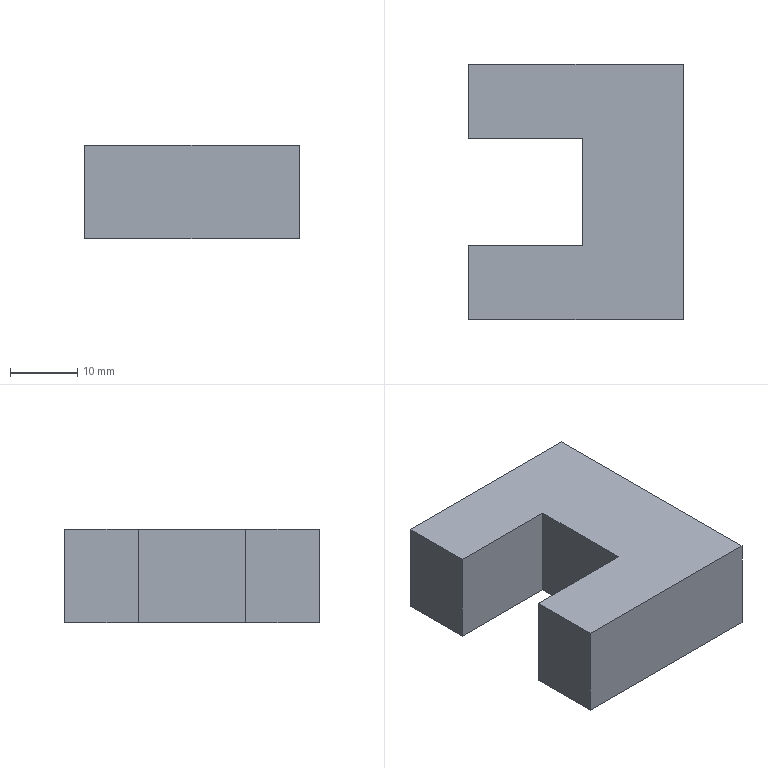Component | SolidWorks | PointedHeadDispensingStopPoint-1 | 1 solid | 18 faces | box 32 x 38 x 14 mm | volume 12816 mm3 | plane 10 | cone 4 | cylinder 4 | commonest cylinder face diameters 4.2 x4
build123d program:
from build123d import *

# Parameters (mm, degrees)
SKETCH1_W             = 32
SKETCH1_H             = 14
EXTRUDE1_DEPTH        = 38
SKETCH3_W             = 17
SKETCH3_H             = 16
CUT_EXTRUDE1_DEPTH    = 52.614
M5_TAPPED_HOLE1_D     = 4.2
M5_TAPPED_HOLE1_DEPTH = 14
M5_TAPPED_HOLE1_TIP   = 1.262


with BuildPart() as part:
    # Sketch1 → Extrude1 (new body)
    with BuildSketch(Plane(origin=(0, 0, 0), x_dir=(1, 0, 0), z_dir=(0, 1, 0))):
        with Locations((16, -7)):
            Rectangle(SKETCH1_W, SKETCH1_H)
    extrude(amount=EXTRUDE1_DEPTH)

    # Sketch3 → Cut-Extrude1 (cut, through all)
    with BuildSketch(Plane.XY.offset(14)):
        with Locations((8.5, 19)):
            Rectangle(SKETCH3_W, SKETCH3_H)
    extrude(amount=-CUT_EXTRUDE1_DEPTH, mode=Mode.SUBTRACT)

    # M5 Tapped Hole1
    with Locations(Plane(origin=(32, 0, 0), x_dir=(0, 0, -1), z_dir=(1, 0, 0))):
        with Locations((-7, 5), (-7, 33)):
            Hole(M5_TAPPED_HOLE1_D / 2, depth=M5_TAPPED_HOLE1_DEPTH)
            with Locations((0, 0, -(M5_TAPPED_HOLE1_DEPTH + M5_TAPPED_HOLE1_TIP / 2))):  # 118° drill point
                Cone(0, M5_TAPPED_HOLE1_D / 2, M5_TAPPED_HOLE1_TIP, mode=Mode.SUBTRACT)


solid = part.part

# Placed as in the assembly
solid = solid.moved(Location((-19.083, 26.872, -124.387), (0, 0, 0)))
STEP:
#1=COLOUR_RGB('',0.7922,0.8196,0.9333);
#2=FILL_AREA_STYLE_COLOUR('',#1);
#3=FILL_AREA_STYLE('',(#2));
#4=SURFACE_STYLE_FILL_AREA(#3);
#5=SURFACE_SIDE_STYLE('',(#4));
#6=SURFACE_STYLE_USAGE(.BOTH.,#5);
#7=PRESENTATION_STYLE_ASSIGNMENT((#6));
#8=CARTESIAN_POINT('',(-0.09232,1.255,-4.622));
#9=VERTEX_POINT('',#8);
#10=CARTESIAN_POINT('',(-0.04264,1.255,-4.704));
#11=VERTEX_POINT('',#10);
#12=CARTESIAN_POINT('',(-0.04264,1.255,-4.704));
#13=DIRECTION('',(0.515,0.,-0.8572));
#14=VECTOR('',#13,39.37);
#15=LINE('',#12,#14);
#16=EDGE_CURVE('',#9,#11,#15,.T.);
#17=ORIENTED_EDGE('',*,*,#16,.F.);
#18=CARTESIAN_POINT('',(-0.04264,1.255,-4.539));
#19=VERTEX_POINT('',#18);
#20=CARTESIAN_POINT('',(-0.04264,1.255,-4.539));
#21=DIRECTION('',(0.515,0.,0.8572));
#22=VECTOR('',#21,39.37);
#23=LINE('',#20,#22);
#24=EDGE_CURVE('',#9,#19,#23,.T.);
#25=ORIENTED_EDGE('',*,*,#24,.T.);
#26=CARTESIAN_POINT('',(-0.04264,1.255,-4.622));
#27=DIRECTION('',(1.,0.,0.));
#28=DIRECTION('',(0.,0.,-1.));
#29=AXIS2_PLACEMENT_3D('',#26,#27,#28);
#30=CIRCLE('',#29,0.08268);
#31=EDGE_CURVE('',#19,#11,#30,.T.);
#32=ORIENTED_EDGE('',*,*,#31,.T.);
#33=EDGE_LOOP('',(#17,#25,#32));
#34=FACE_OUTER_BOUND('',#33,.T.);
#35=CARTESIAN_POINT('',(-0.04264,1.255,-4.622));
#36=DIRECTION('',(1.,0.,0.));
#37=DIRECTION('',(0.,0.,-1.));
#38=AXIS2_PLACEMENT_3D('',#35,#36,#37);
#39=CONICAL_SURFACE('',#38,0.08268,1.03);
#40=ADVANCED_FACE('',(#34),#39,.F.);
#41=ORIENTED_EDGE('',*,*,#31,.F.);
#42=CARTESIAN_POINT('',(0.5085,1.255,-4.539));
#43=VERTEX_POINT('',#42);
#44=CARTESIAN_POINT('',(0.5085,1.255,-4.539));
#45=DIRECTION('',(1.,0.,0.));
#46=VECTOR('',#45,39.37);
#47=LINE('',#44,#46);
#48=EDGE_CURVE('',#19,#43,#47,.T.);
#49=ORIENTED_EDGE('',*,*,#48,.T.);
#50=CARTESIAN_POINT('',(0.5085,1.255,-4.704));
#51=VERTEX_POINT('',#50);
#52=CARTESIAN_POINT('',(0.5085,1.255,-4.622));
#53=DIRECTION('',(1.,0.,0.));
#54=DIRECTION('',(0.,0.,-1.));
#55=AXIS2_PLACEMENT_3D('',#52,#53,#54);
#56=CIRCLE('',#55,0.08268);
#57=EDGE_CURVE('',#43,#51,#56,.T.);
#58=ORIENTED_EDGE('',*,*,#57,.T.);
#59=CARTESIAN_POINT('',(0.5085,1.255,-4.704));
#60=DIRECTION('',(1.,0.,0.));
#61=VECTOR('',#60,39.37);
#62=LINE('',#59,#61);
#63=EDGE_CURVE('',#11,#51,#62,.T.);
#64=ORIENTED_EDGE('',*,*,#63,.F.);
#65=EDGE_LOOP('',(#41,#49,#58,#64));
#66=FACE_OUTER_BOUND('',#65,.T.);
#67=CARTESIAN_POINT('',(0.5085,1.255,-4.622));
#68=DIRECTION('',(1.,0.,0.));
#69=DIRECTION('',(0.,0.,-1.));
#70=AXIS2_PLACEMENT_3D('',#67,#68,#69);
#71=CYLINDRICAL_SURFACE('',#70,0.08268);
#72=ADVANCED_FACE('',(#66),#71,.F.);
#73=CARTESIAN_POINT('',(-0.09232,2.357,-4.622));
#74=VERTEX_POINT('',#73);
#75=CARTESIAN_POINT('',(-0.04264,2.357,-4.704));
#76=VERTEX_POINT('',#75);
#77=CARTESIAN_POINT('',(-0.04264,2.357,-4.704));
#78=DIRECTION('',(0.515,0.,-0.8572));
#79=VECTOR('',#78,39.37);
#80=LINE('',#77,#79);
#81=EDGE_CURVE('',#74,#76,#80,.T.);
#82=ORIENTED_EDGE('',*,*,#81,.F.);
#83=CARTESIAN_POINT('',(-0.04264,2.357,-4.539));
#84=VERTEX_POINT('',#83);
#85=CARTESIAN_POINT('',(-0.04264,2.357,-4.539));
#86=DIRECTION('',(0.515,0.,0.8572));
#87=VECTOR('',#86,39.37);
#88=LINE('',#85,#87);
#89=EDGE_CURVE('',#74,#84,#88,.T.);
#90=ORIENTED_EDGE('',*,*,#89,.T.);
#91=CARTESIAN_POINT('',(-0.04264,2.357,-4.622));
#92=DIRECTION('',(1.,0.,0.));
#93=DIRECTION('',(0.,0.,-1.));
#94=AXIS2_PLACEMENT_3D('',#91,#92,#93);
#95=CIRCLE('',#94,0.08268);
#96=EDGE_CURVE('',#84,#76,#95,.T.);
#97=ORIENTED_EDGE('',*,*,#96,.T.);
#98=EDGE_LOOP('',(#82,#90,#97));
#99=FACE_OUTER_BOUND('',#98,.T.);
#100=CARTESIAN_POINT('',(-0.04264,2.357,-4.622));
#101=DIRECTION('',(1.,0.,0.));
#102=DIRECTION('',(0.,0.,-1.));
#103=AXIS2_PLACEMENT_3D('',#100,#101,#102);
#104=CONICAL_SURFACE('',#103,0.08268,1.03);
#105=ADVANCED_FACE('',(#99),#104,.F.);
#106=ORIENTED_EDGE('',*,*,#96,.F.);
#107=CARTESIAN_POINT('',(0.5085,2.357,-4.539));
#108=VERTEX_POINT('',#107);
#109=CARTESIAN_POINT('',(0.5085,2.357,-4.539));
#110=DIRECTION('',(1.,0.,0.));
#111=VECTOR('',#110,39.37);
#112=LINE('',#109,#111);
#113=EDGE_CURVE('',#84,#108,#112,.T.);
#114=ORIENTED_EDGE('',*,*,#113,.T.);
#115=CARTESIAN_POINT('',(0.5085,2.357,-4.704));
#116=VERTEX_POINT('',#115);
#117=CARTESIAN_POINT('',(0.5085,2.357,-4.622));
#118=DIRECTION('',(1.,0.,0.));
#119=DIRECTION('',(0.,0.,-1.));
#120=AXIS2_PLACEMENT_3D('',#117,#118,#119);
#121=CIRCLE('',#120,0.08268);
#122=EDGE_CURVE('',#108,#116,#121,.T.);
#123=ORIENTED_EDGE('',*,*,#122,.T.);
#124=CARTESIAN_POINT('',(0.5085,2.357,-4.704));
#125=DIRECTION('',(1.,0.,0.));
#126=VECTOR('',#125,39.37);
#127=LINE('',#124,#126);
#128=EDGE_CURVE('',#76,#116,#127,.T.);
#129=ORIENTED_EDGE('',*,*,#128,.F.);
#130=EDGE_LOOP('',(#106,#114,#123,#129));
#131=FACE_OUTER_BOUND('',#130,.T.);
#132=CARTESIAN_POINT('',(0.5085,2.357,-4.622));
#133=DIRECTION('',(1.,0.,0.));
#134=DIRECTION('',(0.,0.,-1.));
#135=AXIS2_PLACEMENT_3D('',#132,#133,#134);
#136=CYLINDRICAL_SURFACE('',#135,0.08268);
#137=ADVANCED_FACE('',(#131),#136,.F.);
#138=CARTESIAN_POINT('',(-0.7513,1.491,-4.346));
#139=VERTEX_POINT('',#138);
#140=CARTESIAN_POINT('',(-0.7513,1.058,-4.346));
#141=VERTEX_POINT('',#140);
#142=CARTESIAN_POINT('',(-0.7513,2.554,-4.346));
#143=DIRECTION('',(0.,-1.,0.));
#144=VECTOR('',#143,39.37);
#145=LINE('',#142,#144);
#146=EDGE_CURVE('',#139,#141,#145,.T.);
#147=ORIENTED_EDGE('',*,*,#146,.F.);
#148=CARTESIAN_POINT('',(-0.7513,1.491,-4.897));
#149=VERTEX_POINT('',#148);
#150=CARTESIAN_POINT('',(-0.7513,1.491,-4.897));
#151=DIRECTION('',(0.,0.,1.));
#152=VECTOR('',#151,39.37);
#153=LINE('',#150,#152);
#154=EDGE_CURVE('',#149,#139,#153,.T.);
#155=ORIENTED_EDGE('',*,*,#154,.F.);
#156=CARTESIAN_POINT('',(-0.7513,1.058,-4.897));
#157=VERTEX_POINT('',#156);
#158=CARTESIAN_POINT('',(-0.7513,2.554,-4.897));
#159=DIRECTION('',(0.,-1.,0.));
#160=VECTOR('',#159,39.37);
#161=LINE('',#158,#160);
#162=EDGE_CURVE('',#149,#157,#161,.T.);
#163=ORIENTED_EDGE('',*,*,#162,.T.);
#164=CARTESIAN_POINT('',(-0.7513,1.058,-4.897));
#165=DIRECTION('',(0.,0.,1.));
#166=VECTOR('',#165,39.37);
#167=LINE('',#164,#166);
#168=EDGE_CURVE('',#157,#141,#167,.T.);
#169=ORIENTED_EDGE('',*,*,#168,.T.);
#170=EDGE_LOOP('',(#147,#155,#163,#169));
#171=FACE_OUTER_BOUND('',#170,.T.);
#172=CARTESIAN_POINT('',(-0.7513,2.554,-4.897));
#173=DIRECTION('',(1.,0.,-0.));
#174=DIRECTION('',(-0.,0.,-1.));
#175=AXIS2_PLACEMENT_3D('',#172,#173,#174);
#176=PLANE('',#175);
#177=ADVANCED_FACE('',(#171),#176,.F.);
#178=CARTESIAN_POINT('',(-0.7513,2.554,-4.897));
#179=VERTEX_POINT('',#178);
#180=CARTESIAN_POINT('',(-0.7513,2.121,-4.897));
#181=VERTEX_POINT('',#180);
#182=CARTESIAN_POINT('',(-0.7513,2.554,-4.897));
#183=DIRECTION('',(0.,-1.,0.));
#184=VECTOR('',#183,39.37);
#185=LINE('',#182,#184);
#186=EDGE_CURVE('',#179,#181,#185,.T.);
#187=ORIENTED_EDGE('',*,*,#186,.T.);
#188=CARTESIAN_POINT('',(-0.7513,2.121,-4.346));
#189=VERTEX_POINT('',#188);
#190=CARTESIAN_POINT('',(-0.7513,2.121,-4.897));
#191=DIRECTION('',(0.,0.,1.));
#192=VECTOR('',#191,39.37);
#193=LINE('',#190,#192);
#194=EDGE_CURVE('',#181,#189,#193,.T.);
#195=ORIENTED_EDGE('',*,*,#194,.T.);
#196=CARTESIAN_POINT('',(-0.7513,2.554,-4.346));
#197=VERTEX_POINT('',#196);
#198=CARTESIAN_POINT('',(-0.7513,2.554,-4.346));
#199=DIRECTION('',(0.,-1.,0.));
#200=VECTOR('',#199,39.37);
#201=LINE('',#198,#200);
#202=EDGE_CURVE('',#197,#189,#201,.T.);
#203=ORIENTED_EDGE('',*,*,#202,.F.);
#204=CARTESIAN_POINT('',(-0.7513,2.554,-4.897));
#205=DIRECTION('',(0.,0.,1.));
#206=VECTOR('',#205,39.37);
#207=LINE('',#204,#206);
#208=EDGE_CURVE('',#179,#197,#207,.T.);
#209=ORIENTED_EDGE('',*,*,#208,.F.);
#210=EDGE_LOOP('',(#187,#195,#203,#209));
#211=FACE_OUTER_BOUND('',#210,.T.);
#212=CARTESIAN_POINT('',(-0.7513,2.554,-4.897));
#213=DIRECTION('',(1.,0.,-0.));
#214=DIRECTION('',(-0.,0.,-1.));
#215=AXIS2_PLACEMENT_3D('',#212,#213,#214);
#216=PLANE('',#215);
#217=ADVANCED_FACE('',(#211),#216,.F.);
#218=CARTESIAN_POINT('',(-0.08201,1.491,-4.346));
#219=VERTEX_POINT('',#218);
#220=CARTESIAN_POINT('',(-0.08201,2.121,-4.346));
#221=VERTEX_POINT('',#220);
#222=CARTESIAN_POINT('',(-0.08201,2.121,-4.346));
#223=DIRECTION('',(-0.,1.,0.));
#224=VECTOR('',#223,39.37);
#225=LINE('',#222,#224);
#226=EDGE_CURVE('',#219,#221,#225,.T.);
#227=ORIENTED_EDGE('',*,*,#226,.F.);
#228=CARTESIAN_POINT('',(-0.08201,1.491,-4.346));
#229=DIRECTION('',(1.,0.,0.));
#230=VECTOR('',#229,39.37);
#231=LINE('',#228,#230);
#232=EDGE_CURVE('',#139,#219,#231,.T.);
#233=ORIENTED_EDGE('',*,*,#232,.F.);
#234=ORIENTED_EDGE('',*,*,#146,.T.);
#235=CARTESIAN_POINT('',(0.5085,1.058,-4.346));
#236=VERTEX_POINT('',#235);
#237=CARTESIAN_POINT('',(-0.7513,1.058,-4.346));
#238=DIRECTION('',(1.,0.,0.));
#239=VECTOR('',#238,39.37);
#240=LINE('',#237,#239);
#241=EDGE_CURVE('',#141,#236,#240,.T.);
#242=ORIENTED_EDGE('',*,*,#241,.T.);
#243=CARTESIAN_POINT('',(0.5085,2.554,-4.346));
#244=VERTEX_POINT('',#243);
#245=CARTESIAN_POINT('',(0.5085,2.554,-4.346));
#246=DIRECTION('',(0.,-1.,0.));
#247=VECTOR('',#246,39.37);
#248=LINE('',#245,#247);
#249=EDGE_CURVE('',#244,#236,#248,.T.);
#250=ORIENTED_EDGE('',*,*,#249,.F.);
#251=CARTESIAN_POINT('',(-0.7513,2.554,-4.346));
#252=DIRECTION('',(1.,0.,0.));
#253=VECTOR('',#252,39.37);
#254=LINE('',#251,#253);
#255=EDGE_CURVE('',#197,#244,#254,.T.);
#256=ORIENTED_EDGE('',*,*,#255,.F.);
#257=ORIENTED_EDGE('',*,*,#202,.T.);
#258=CARTESIAN_POINT('',(-0.08201,2.121,-4.346));
#259=DIRECTION('',(-1.,0.,0.));
#260=VECTOR('',#259,39.37);
#261=LINE('',#258,#260);
#262=EDGE_CURVE('',#221,#189,#261,.T.);
#263=ORIENTED_EDGE('',*,*,#262,.F.);
#264=EDGE_LOOP('',(#227,#233,#234,#242,#250,#256,#257,#263));
#265=FACE_OUTER_BOUND('',#264,.T.);
#266=CARTESIAN_POINT('',(-0.7513,2.554,-4.346));
#267=DIRECTION('',(0.,0.,-1.));
#268=DIRECTION('',(-1.,0.,0.));
#269=AXIS2_PLACEMENT_3D('',#266,#267,#268);
#270=PLANE('',#269);
#271=ADVANCED_FACE('',(#265),#270,.F.);
#272=CARTESIAN_POINT('',(0.5085,1.255,-4.622));
#273=DIRECTION('',(1.,0.,0.));
#274=DIRECTION('',(0.,0.,-1.));
#275=AXIS2_PLACEMENT_3D('',#272,#273,#274);
#276=CIRCLE('',#275,0.08268);
#277=EDGE_CURVE('',#51,#43,#276,.T.);
#278=ORIENTED_EDGE('',*,*,#277,.F.);
#279=ORIENTED_EDGE('',*,*,#57,.F.);
#280=EDGE_LOOP('',(#278,#279));
#281=FACE_BOUND('',#280,.T.);
#282=CARTESIAN_POINT('',(0.5085,2.357,-4.622));
#283=DIRECTION('',(1.,0.,0.));
#284=DIRECTION('',(0.,0.,-1.));
#285=AXIS2_PLACEMENT_3D('',#282,#283,#284);
#286=CIRCLE('',#285,0.08268);
#287=EDGE_CURVE('',#116,#108,#286,.T.);
#288=ORIENTED_EDGE('',*,*,#287,.F.);
#289=ORIENTED_EDGE('',*,*,#122,.F.);
#290=EDGE_LOOP('',(#288,#289));
#291=FACE_BOUND('',#290,.T.);
#292=CARTESIAN_POINT('',(0.5085,1.058,-4.897));
#293=VERTEX_POINT('',#292);
#294=CARTESIAN_POINT('',(0.5085,1.058,-4.897));
#295=DIRECTION('',(0.,0.,-1.));
#296=VECTOR('',#295,39.37);
#297=LINE('',#294,#296);
#298=EDGE_CURVE('',#236,#293,#297,.T.);
#299=ORIENTED_EDGE('',*,*,#298,.T.);
#300=CARTESIAN_POINT('',(0.5085,2.554,-4.897));
#301=VERTEX_POINT('',#300);
#302=CARTESIAN_POINT('',(0.5085,2.554,-4.897));
#303=DIRECTION('',(0.,-1.,0.));
#304=VECTOR('',#303,39.37);
#305=LINE('',#302,#304);
#306=EDGE_CURVE('',#301,#293,#305,.T.);
#307=ORIENTED_EDGE('',*,*,#306,.F.);
#308=CARTESIAN_POINT('',(0.5085,2.554,-4.897));
#309=DIRECTION('',(0.,0.,-1.));
#310=VECTOR('',#309,39.37);
#311=LINE('',#308,#310);
#312=EDGE_CURVE('',#244,#301,#311,.T.);
#313=ORIENTED_EDGE('',*,*,#312,.F.);
#314=ORIENTED_EDGE('',*,*,#249,.T.);
#315=EDGE_LOOP('',(#299,#307,#313,#314));
#316=FACE_OUTER_BOUND('',#315,.T.);
#317=CARTESIAN_POINT('',(0.5085,2.554,-4.897));
#318=DIRECTION('',(-1.,0.,0.));
#319=DIRECTION('',(0.,0.,1.));
#320=AXIS2_PLACEMENT_3D('',#317,#318,#319);
#321=PLANE('',#320);
#322=ADVANCED_FACE('',(#281,#291,#316),#321,.F.);
#323=ORIENTED_EDGE('',*,*,#162,.F.);
#324=CARTESIAN_POINT('',(-0.08201,1.491,-4.897));
#325=VERTEX_POINT('',#324);
#326=CARTESIAN_POINT('',(-0.08201,1.491,-4.897));
#327=DIRECTION('',(1.,0.,0.));
#328=VECTOR('',#327,39.37);
#329=LINE('',#326,#328);
#330=EDGE_CURVE('',#149,#325,#329,.T.);
#331=ORIENTED_EDGE('',*,*,#330,.T.);
#332=CARTESIAN_POINT('',(-0.08201,2.121,-4.897));
#333=VERTEX_POINT('',#332);
#334=CARTESIAN_POINT('',(-0.08201,2.121,-4.897));
#335=DIRECTION('',(-0.,1.,0.));
#336=VECTOR('',#335,39.37);
#337=LINE('',#334,#336);
#338=EDGE_CURVE('',#325,#333,#337,.T.);
#339=ORIENTED_EDGE('',*,*,#338,.T.);
#340=CARTESIAN_POINT('',(-0.08201,2.121,-4.897));
#341=DIRECTION('',(-1.,0.,0.));
#342=VECTOR('',#341,39.37);
#343=LINE('',#340,#342);
#344=EDGE_CURVE('',#333,#181,#343,.T.);
#345=ORIENTED_EDGE('',*,*,#344,.T.);
#346=ORIENTED_EDGE('',*,*,#186,.F.);
#347=CARTESIAN_POINT('',(-0.7513,2.554,-4.897));
#348=DIRECTION('',(-1.,0.,0.));
#349=VECTOR('',#348,39.37);
#350=LINE('',#347,#349);
#351=EDGE_CURVE('',#301,#179,#350,.T.);
#352=ORIENTED_EDGE('',*,*,#351,.F.);
#353=ORIENTED_EDGE('',*,*,#306,.T.);
#354=CARTESIAN_POINT('',(-0.7513,1.058,-4.897));
#355=DIRECTION('',(-1.,0.,0.));
#356=VECTOR('',#355,39.37);
#357=LINE('',#354,#356);
#358=EDGE_CURVE('',#293,#157,#357,.T.);
#359=ORIENTED_EDGE('',*,*,#358,.T.);
#360=EDGE_LOOP('',(#323,#331,#339,#345,#346,#352,#353,#359));
#361=FACE_OUTER_BOUND('',#360,.T.);
#362=CARTESIAN_POINT('',(-0.7513,2.554,-4.897));
#363=DIRECTION('',(0.,0.,1.));
#364=DIRECTION('',(1.,0.,0.));
#365=AXIS2_PLACEMENT_3D('',#362,#363,#364);
#366=PLANE('',#365);
#367=ADVANCED_FACE('',(#361),#366,.F.);
#368=ORIENTED_EDGE('',*,*,#208,.T.);
#369=ORIENTED_EDGE('',*,*,#255,.T.);
#370=ORIENTED_EDGE('',*,*,#312,.T.);
#371=ORIENTED_EDGE('',*,*,#351,.T.);
#372=EDGE_LOOP('',(#368,#369,#370,#371));
#373=FACE_OUTER_BOUND('',#372,.T.);
#374=CARTESIAN_POINT('',(-0.7513,2.554,-4.346));
#375=DIRECTION('',(0.,1.,0.));
#376=DIRECTION('',(0.,0.,1.));
#377=AXIS2_PLACEMENT_3D('',#374,#375,#376);
#378=PLANE('',#377);
#379=ADVANCED_FACE('',(#373),#378,.T.);
#380=ORIENTED_EDGE('',*,*,#168,.F.);
#381=ORIENTED_EDGE('',*,*,#358,.F.);
#382=ORIENTED_EDGE('',*,*,#298,.F.);
#383=ORIENTED_EDGE('',*,*,#241,.F.);
#384=EDGE_LOOP('',(#380,#381,#382,#383));
#385=FACE_OUTER_BOUND('',#384,.T.);
#386=CARTESIAN_POINT('',(-0.7513,1.058,-4.346));
#387=DIRECTION('',(0.,1.,0.));
#388=DIRECTION('',(0.,0.,1.));
#389=AXIS2_PLACEMENT_3D('',#386,#387,#388);
#390=PLANE('',#389);
#391=ADVANCED_FACE('',(#385),#390,.F.);
#392=ORIENTED_EDGE('',*,*,#226,.T.);
#393=CARTESIAN_POINT('',(-0.08201,2.121,-4.897));
#394=DIRECTION('',(0.,0.,1.));
#395=VECTOR('',#394,39.37);
#396=LINE('',#393,#395);
#397=EDGE_CURVE('',#333,#221,#396,.T.);
#398=ORIENTED_EDGE('',*,*,#397,.F.);
#399=ORIENTED_EDGE('',*,*,#338,.F.);
#400=CARTESIAN_POINT('',(-0.08201,1.491,-4.897));
#401=DIRECTION('',(0.,0.,1.));
#402=VECTOR('',#401,39.37);
#403=LINE('',#400,#402);
#404=EDGE_CURVE('',#325,#219,#403,.T.);
#405=ORIENTED_EDGE('',*,*,#404,.T.);
#406=EDGE_LOOP('',(#392,#398,#399,#405));
#407=FACE_OUTER_BOUND('',#406,.T.);
#408=CARTESIAN_POINT('',(-0.08201,2.121,-4.897));
#409=DIRECTION('',(1.,0.,0.));
#410=DIRECTION('',(-0.,1.,0.));
#411=AXIS2_PLACEMENT_3D('',#408,#409,#410);
#412=PLANE('',#411);
#413=ADVANCED_FACE('',(#407),#412,.F.);
#414=ORIENTED_EDGE('',*,*,#232,.T.);
#415=ORIENTED_EDGE('',*,*,#404,.F.);
#416=ORIENTED_EDGE('',*,*,#330,.F.);
#417=ORIENTED_EDGE('',*,*,#154,.T.);
#418=EDGE_LOOP('',(#414,#415,#416,#417));
#419=FACE_OUTER_BOUND('',#418,.T.);
#420=CARTESIAN_POINT('',(-0.08201,1.491,-4.897));
#421=DIRECTION('',(0.,-1.,0.));
#422=DIRECTION('',(0.,0.,-1.));
#423=AXIS2_PLACEMENT_3D('',#420,#421,#422);
#424=PLANE('',#423);
#425=ADVANCED_FACE('',(#419),#424,.F.);
#426=ORIENTED_EDGE('',*,*,#262,.T.);
#427=ORIENTED_EDGE('',*,*,#194,.F.);
#428=ORIENTED_EDGE('',*,*,#344,.F.);
#429=ORIENTED_EDGE('',*,*,#397,.T.);
#430=EDGE_LOOP('',(#426,#427,#428,#429));
#431=FACE_OUTER_BOUND('',#430,.T.);
#432=CARTESIAN_POINT('',(-0.08201,2.121,-4.897));
#433=DIRECTION('',(0.,1.,0.));
#434=DIRECTION('',(0.,0.,1.));
#435=AXIS2_PLACEMENT_3D('',#432,#433,#434);
#436=PLANE('',#435);
#437=ADVANCED_FACE('',(#431),#436,.F.);
#438=ORIENTED_EDGE('',*,*,#113,.F.);
#439=CARTESIAN_POINT('',(-0.04264,2.357,-4.622));
#440=DIRECTION('',(1.,0.,0.));
#441=DIRECTION('',(0.,0.,-1.));
#442=AXIS2_PLACEMENT_3D('',#439,#440,#441);
#443=CIRCLE('',#442,0.08268);
#444=EDGE_CURVE('',#76,#84,#443,.T.);
#445=ORIENTED_EDGE('',*,*,#444,.F.);
#446=ORIENTED_EDGE('',*,*,#128,.T.);
#447=ORIENTED_EDGE('',*,*,#287,.T.);
#448=EDGE_LOOP('',(#438,#445,#446,#447));
#449=FACE_OUTER_BOUND('',#448,.T.);
#450=CARTESIAN_POINT('',(0.5085,2.357,-4.622));
#451=DIRECTION('',(1.,0.,0.));
#452=DIRECTION('',(0.,0.,-1.));
#453=AXIS2_PLACEMENT_3D('',#450,#451,#452);
#454=CYLINDRICAL_SURFACE('',#453,0.08268);
#455=ADVANCED_FACE('',(#449),#454,.F.);
#456=ORIENTED_EDGE('',*,*,#89,.F.);
#457=ORIENTED_EDGE('',*,*,#81,.T.);
#458=ORIENTED_EDGE('',*,*,#444,.T.);
#459=EDGE_LOOP('',(#456,#457,#458));
#460=FACE_OUTER_BOUND('',#459,.T.);
#461=CARTESIAN_POINT('',(-0.04264,2.357,-4.622));
#462=DIRECTION('',(1.,0.,0.));
#463=DIRECTION('',(0.,0.,-1.));
#464=AXIS2_PLACEMENT_3D('',#461,#462,#463);
#465=CONICAL_SURFACE('',#464,0.08268,1.03);
#466=ADVANCED_FACE('',(#460),#465,.F.);
#467=ORIENTED_EDGE('',*,*,#48,.F.);
#468=CARTESIAN_POINT('',(-0.04264,1.255,-4.622));
#469=DIRECTION('',(1.,0.,0.));
#470=DIRECTION('',(0.,0.,-1.));
#471=AXIS2_PLACEMENT_3D('',#468,#469,#470);
#472=CIRCLE('',#471,0.08268);
#473=EDGE_CURVE('',#11,#19,#472,.T.);
#474=ORIENTED_EDGE('',*,*,#473,.F.);
#475=ORIENTED_EDGE('',*,*,#63,.T.);
#476=ORIENTED_EDGE('',*,*,#277,.T.);
#477=EDGE_LOOP('',(#467,#474,#475,#476));
#478=FACE_OUTER_BOUND('',#477,.T.);
#479=CARTESIAN_POINT('',(0.5085,1.255,-4.622));
#480=DIRECTION('',(1.,0.,0.));
#481=DIRECTION('',(0.,0.,-1.));
#482=AXIS2_PLACEMENT_3D('',#479,#480,#481);
#483=CYLINDRICAL_SURFACE('',#482,0.08268);
#484=ADVANCED_FACE('',(#478),#483,.F.);
#485=ORIENTED_EDGE('',*,*,#24,.F.);
#486=ORIENTED_EDGE('',*,*,#16,.T.);
#487=ORIENTED_EDGE('',*,*,#473,.T.);
#488=EDGE_LOOP('',(#485,#486,#487));
#489=FACE_OUTER_BOUND('',#488,.T.);
#490=CARTESIAN_POINT('',(-0.04264,1.255,-4.622));
#491=DIRECTION('',(1.,0.,0.));
#492=DIRECTION('',(0.,0.,-1.));
#493=AXIS2_PLACEMENT_3D('',#490,#491,#492);
#494=CONICAL_SURFACE('',#493,0.08268,1.03);
#495=ADVANCED_FACE('',(#489),#494,.F.);
#496=CLOSED_SHELL('',(#40,#72,#105,#137,#177,#217,#271,#322,#367,#379,#391,#413,#425,#437,#455,#466,#484,#495));
#497=MANIFOLD_SOLID_BREP('',#496);
#498=STYLED_ITEM('',(#7),#497);
#499=(LENGTH_UNIT()NAMED_UNIT(*)SI_UNIT($,.METRE.));
#500=LENGTH_MEASURE_WITH_UNIT(LENGTH_MEASURE(0.0254),#499);
#501=DIMENSIONAL_EXPONENTS(1.,0.,0.,0.,0.,0.,0.);
#502=(CONVERSION_BASED_UNIT('',#500)LENGTH_UNIT()NAMED_UNIT(#501));
#503=UNCERTAINTY_MEASURE_WITH_UNIT(LENGTH_MEASURE(0.00001),#502,'','');
#504=(NAMED_UNIT(*)PLANE_ANGLE_UNIT()SI_UNIT($,.RADIAN.));
#505=(NAMED_UNIT(*)SI_UNIT($,.STERADIAN.)SOLID_ANGLE_UNIT());
#506=(GEOMETRIC_REPRESENTATION_CONTEXT(3)GLOBAL_UNCERTAINTY_ASSIGNED_CONTEXT((#503))GLOBAL_UNIT_ASSIGNED_CONTEXT((#502,#504,#505))REPRESENTATION_CONTEXT('',''));
#507=MECHANICAL_DESIGN_GEOMETRIC_PRESENTATION_REPRESENTATION('',(#498),#506);
#508=CARTESIAN_POINT('',(0.,0.,0.));
#509=DIRECTION('',(0.,0.,1.));
#510=DIRECTION('',(1.,0.,0.));
#511=AXIS2_PLACEMENT_3D('',#508,#509,#510);
#512=(LENGTH_UNIT()NAMED_UNIT(*)SI_UNIT($,.METRE.));
#513=LENGTH_MEASURE_WITH_UNIT(LENGTH_MEASURE(0.0254),#512);
#514=DIMENSIONAL_EXPONENTS(1.,0.,0.,0.,0.,0.,0.);
#515=(CONVERSION_BASED_UNIT('',#513)LENGTH_UNIT()NAMED_UNIT(#514));
#516=UNCERTAINTY_MEASURE_WITH_UNIT(LENGTH_MEASURE(0.00001),#515,'','');
#517=(NAMED_UNIT(*)PLANE_ANGLE_UNIT()SI_UNIT($,.RADIAN.));
#518=(NAMED_UNIT(*)SI_UNIT($,.STERADIAN.)SOLID_ANGLE_UNIT());
#519=(GEOMETRIC_REPRESENTATION_CONTEXT(3)GLOBAL_UNCERTAINTY_ASSIGNED_CONTEXT((#516))GLOBAL_UNIT_ASSIGNED_CONTEXT((#515,#517,#518))REPRESENTATION_CONTEXT('',''));
#520=ADVANCED_BREP_SHAPE_REPRESENTATION('',(#497,#511),#519);
#521=PRESENTATION_LAYER_ASSIGNMENT('','',(#498));